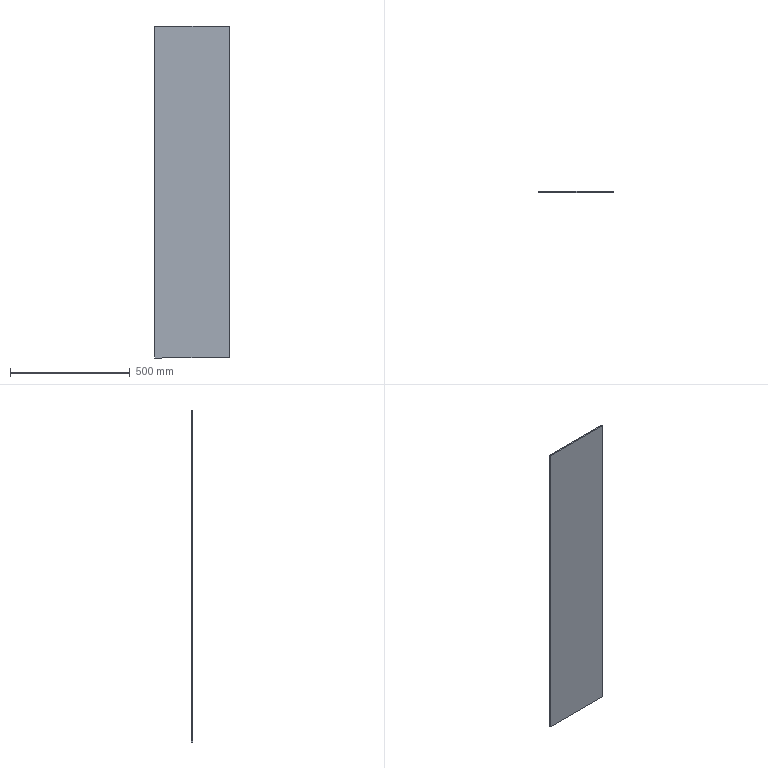Component | SolidWorks | GlassDoorAssembly-1_TemperedGlass5mm-2 | 1 solid | 6 faces | box 310 x 5 x 1385 mm | volume 2146750 mm3 | plane 6
STEP:
#1=COLOUR_RGB('',0.7922,0.8196,0.9333);
#2=FILL_AREA_STYLE_COLOUR('',#1);
#3=FILL_AREA_STYLE('',(#2));
#4=SURFACE_STYLE_FILL_AREA(#3);
#5=SURFACE_SIDE_STYLE('',(#4));
#6=SURFACE_STYLE_USAGE(.BOTH.,#5);
#7=PRESENTATION_STYLE_ASSIGNMENT((#6));
#8=CARTESIAN_POINT('',(-1.716,-19.846,-58.701));
#9=VERTEX_POINT('',#8);
#10=CARTESIAN_POINT('',(-13.92,-19.846,-58.701));
#11=VERTEX_POINT('',#10);
#12=CARTESIAN_POINT('',(-13.92,-19.846,-58.701));
#13=DIRECTION('',(-1.,-0.,-0.));
#14=VECTOR('',#13,39.37);
#15=LINE('',#12,#14);
#16=EDGE_CURVE('',#9,#11,#15,.T.);
#17=ORIENTED_EDGE('',*,*,#16,.F.);
#18=CARTESIAN_POINT('',(-1.716,-20.042,-58.701));
#19=VERTEX_POINT('',#18);
#20=CARTESIAN_POINT('',(-1.716,-20.042,-58.701));
#21=DIRECTION('',(-0.,1.,0.));
#22=VECTOR('',#21,39.37);
#23=LINE('',#20,#22);
#24=EDGE_CURVE('',#19,#9,#23,.T.);
#25=ORIENTED_EDGE('',*,*,#24,.F.);
#26=CARTESIAN_POINT('',(-13.92,-20.042,-58.701));
#27=VERTEX_POINT('',#26);
#28=CARTESIAN_POINT('',(-13.92,-20.042,-58.701));
#29=DIRECTION('',(-1.,-0.,-0.));
#30=VECTOR('',#29,39.37);
#31=LINE('',#28,#30);
#32=EDGE_CURVE('',#19,#27,#31,.T.);
#33=ORIENTED_EDGE('',*,*,#32,.T.);
#34=CARTESIAN_POINT('',(-13.92,-20.042,-58.701));
#35=DIRECTION('',(-0.,1.,0.));
#36=VECTOR('',#35,39.37);
#37=LINE('',#34,#36);
#38=EDGE_CURVE('',#27,#11,#37,.T.);
#39=ORIENTED_EDGE('',*,*,#38,.T.);
#40=EDGE_LOOP('',(#17,#25,#33,#39));
#41=FACE_OUTER_BOUND('',#40,.T.);
#42=CARTESIAN_POINT('',(-13.92,-20.042,-58.701));
#43=DIRECTION('',(0.,0.,-1.));
#44=DIRECTION('',(0.,-1.,-0.));
#45=AXIS2_PLACEMENT_3D('',#42,#43,#44);
#46=PLANE('',#45);
#47=ADVANCED_FACE('',(#41),#46,.T.);
#48=CARTESIAN_POINT('',(-1.716,-19.846,-4.173));
#49=VERTEX_POINT('',#48);
#50=CARTESIAN_POINT('',(-1.716,-19.846,-4.173));
#51=DIRECTION('',(0.,0.,-1.));
#52=VECTOR('',#51,39.37);
#53=LINE('',#50,#52);
#54=EDGE_CURVE('',#49,#9,#53,.T.);
#55=ORIENTED_EDGE('',*,*,#54,.F.);
#56=CARTESIAN_POINT('',(-1.716,-20.042,-4.173));
#57=VERTEX_POINT('',#56);
#58=CARTESIAN_POINT('',(-1.716,-20.042,-4.173));
#59=DIRECTION('',(-0.,1.,0.));
#60=VECTOR('',#59,39.37);
#61=LINE('',#58,#60);
#62=EDGE_CURVE('',#57,#49,#61,.T.);
#63=ORIENTED_EDGE('',*,*,#62,.F.);
#64=CARTESIAN_POINT('',(-1.716,-20.042,-4.173));
#65=DIRECTION('',(0.,0.,-1.));
#66=VECTOR('',#65,39.37);
#67=LINE('',#64,#66);
#68=EDGE_CURVE('',#57,#19,#67,.T.);
#69=ORIENTED_EDGE('',*,*,#68,.T.);
#70=ORIENTED_EDGE('',*,*,#24,.T.);
#71=EDGE_LOOP('',(#55,#63,#69,#70));
#72=FACE_OUTER_BOUND('',#71,.T.);
#73=CARTESIAN_POINT('',(-1.716,-20.042,-4.173));
#74=DIRECTION('',(1.,0.,0.));
#75=DIRECTION('',(0.,-1.,-0.));
#76=AXIS2_PLACEMENT_3D('',#73,#74,#75);
#77=PLANE('',#76);
#78=ADVANCED_FACE('',(#72),#77,.T.);
#79=CARTESIAN_POINT('',(-13.92,-19.846,-4.173));
#80=VERTEX_POINT('',#79);
#81=CARTESIAN_POINT('',(-13.92,-19.846,-4.173));
#82=DIRECTION('',(1.,0.,0.));
#83=VECTOR('',#82,39.37);
#84=LINE('',#81,#83);
#85=EDGE_CURVE('',#80,#49,#84,.T.);
#86=ORIENTED_EDGE('',*,*,#85,.F.);
#87=CARTESIAN_POINT('',(-13.92,-20.042,-4.173));
#88=VERTEX_POINT('',#87);
#89=CARTESIAN_POINT('',(-13.92,-20.042,-4.173));
#90=DIRECTION('',(-0.,1.,0.));
#91=VECTOR('',#90,39.37);
#92=LINE('',#89,#91);
#93=EDGE_CURVE('',#88,#80,#92,.T.);
#94=ORIENTED_EDGE('',*,*,#93,.F.);
#95=CARTESIAN_POINT('',(-13.92,-20.042,-4.173));
#96=DIRECTION('',(1.,0.,0.));
#97=VECTOR('',#96,39.37);
#98=LINE('',#95,#97);
#99=EDGE_CURVE('',#88,#57,#98,.T.);
#100=ORIENTED_EDGE('',*,*,#99,.T.);
#101=ORIENTED_EDGE('',*,*,#62,.T.);
#102=EDGE_LOOP('',(#86,#94,#100,#101));
#103=FACE_OUTER_BOUND('',#102,.T.);
#104=CARTESIAN_POINT('',(-13.92,-20.042,-4.173));
#105=DIRECTION('',(-0.,-0.,1.));
#106=DIRECTION('',(-0.,1.,0.));
#107=AXIS2_PLACEMENT_3D('',#104,#105,#106);
#108=PLANE('',#107);
#109=ADVANCED_FACE('',(#103),#108,.T.);
#110=CARTESIAN_POINT('',(-13.92,-19.846,-4.173));
#111=DIRECTION('',(-0.,-0.,1.));
#112=VECTOR('',#111,39.37);
#113=LINE('',#110,#112);
#114=EDGE_CURVE('',#11,#80,#113,.T.);
#115=ORIENTED_EDGE('',*,*,#114,.F.);
#116=ORIENTED_EDGE('',*,*,#38,.F.);
#117=CARTESIAN_POINT('',(-13.92,-20.042,-4.173));
#118=DIRECTION('',(-0.,-0.,1.));
#119=VECTOR('',#118,39.37);
#120=LINE('',#117,#119);
#121=EDGE_CURVE('',#27,#88,#120,.T.);
#122=ORIENTED_EDGE('',*,*,#121,.T.);
#123=ORIENTED_EDGE('',*,*,#93,.T.);
#124=EDGE_LOOP('',(#115,#116,#122,#123));
#125=FACE_OUTER_BOUND('',#124,.T.);
#126=CARTESIAN_POINT('',(-13.92,-20.042,-4.173));
#127=DIRECTION('',(-1.,-0.,-0.));
#128=DIRECTION('',(-0.,1.,0.));
#129=AXIS2_PLACEMENT_3D('',#126,#127,#128);
#130=PLANE('',#129);
#131=ADVANCED_FACE('',(#125),#130,.T.);
#132=ORIENTED_EDGE('',*,*,#32,.F.);
#133=ORIENTED_EDGE('',*,*,#68,.F.);
#134=ORIENTED_EDGE('',*,*,#99,.F.);
#135=ORIENTED_EDGE('',*,*,#121,.F.);
#136=EDGE_LOOP('',(#132,#133,#134,#135));
#137=FACE_OUTER_BOUND('',#136,.T.);
#138=CARTESIAN_POINT('',(-1.716,-20.042,-58.701));
#139=DIRECTION('',(-0.,1.,0.));
#140=DIRECTION('',(0.,0.,-1.));
#141=AXIS2_PLACEMENT_3D('',#138,#139,#140);
#142=PLANE('',#141);
#143=ADVANCED_FACE('',(#137),#142,.F.);
#144=ORIENTED_EDGE('',*,*,#16,.T.);
#145=ORIENTED_EDGE('',*,*,#114,.T.);
#146=ORIENTED_EDGE('',*,*,#85,.T.);
#147=ORIENTED_EDGE('',*,*,#54,.T.);
#148=EDGE_LOOP('',(#144,#145,#146,#147));
#149=FACE_OUTER_BOUND('',#148,.T.);
#150=CARTESIAN_POINT('',(-1.716,-19.846,-58.701));
#151=DIRECTION('',(-0.,1.,0.));
#152=DIRECTION('',(0.,0.,-1.));
#153=AXIS2_PLACEMENT_3D('',#150,#151,#152);
#154=PLANE('',#153);
#155=ADVANCED_FACE('',(#149),#154,.T.);
#156=CLOSED_SHELL('',(#47,#78,#109,#131,#143,#155));
#157=MANIFOLD_SOLID_BREP('',#156);
#158=STYLED_ITEM('',(#7),#157);
#159=PRESENTATION_LAYER_ASSIGNMENT('','',(#158));
#160=(LENGTH_UNIT()NAMED_UNIT(*)SI_UNIT($,.METRE.));
#161=LENGTH_MEASURE_WITH_UNIT(LENGTH_MEASURE(0.0254),#160);
#162=DIMENSIONAL_EXPONENTS(1.,0.,0.,0.,0.,0.,0.);
#163=(CONVERSION_BASED_UNIT('',#161)LENGTH_UNIT()NAMED_UNIT(#162));
#164=UNCERTAINTY_MEASURE_WITH_UNIT(LENGTH_MEASURE(0.00001),#163,'','');
#165=(NAMED_UNIT(*)PLANE_ANGLE_UNIT()SI_UNIT($,.RADIAN.));
#166=(NAMED_UNIT(*)SI_UNIT($,.STERADIAN.)SOLID_ANGLE_UNIT());
#167=(GEOMETRIC_REPRESENTATION_CONTEXT(3)GLOBAL_UNCERTAINTY_ASSIGNED_CONTEXT((#164))GLOBAL_UNIT_ASSIGNED_CONTEXT((#163,#165,#166))REPRESENTATION_CONTEXT('',''));
#168=MECHANICAL_DESIGN_GEOMETRIC_PRESENTATION_REPRESENTATION('',(#158),#167);
#169=CARTESIAN_POINT('',(0.,0.,0.));
#170=DIRECTION('',(0.,0.,1.));
#171=DIRECTION('',(1.,0.,0.));
#172=AXIS2_PLACEMENT_3D('',#169,#170,#171);
#173=(LENGTH_UNIT()NAMED_UNIT(*)SI_UNIT($,.METRE.));
#174=LENGTH_MEASURE_WITH_UNIT(LENGTH_MEASURE(0.0254),#173);
#175=DIMENSIONAL_EXPONENTS(1.,0.,0.,0.,0.,0.,0.);
#176=(CONVERSION_BASED_UNIT('',#174)LENGTH_UNIT()NAMED_UNIT(#175));
#177=UNCERTAINTY_MEASURE_WITH_UNIT(LENGTH_MEASURE(0.00001),#176,'','');
#178=(NAMED_UNIT(*)PLANE_ANGLE_UNIT()SI_UNIT($,.RADIAN.));
#179=(NAMED_UNIT(*)SI_UNIT($,.STERADIAN.)SOLID_ANGLE_UNIT());
#180=(GEOMETRIC_REPRESENTATION_CONTEXT(3)GLOBAL_UNCERTAINTY_ASSIGNED_CONTEXT((#177))GLOBAL_UNIT_ASSIGNED_CONTEXT((#176,#178,#179))REPRESENTATION_CONTEXT('',''));
#181=ADVANCED_BREP_SHAPE_REPRESENTATION('',(#157,#172),#180);